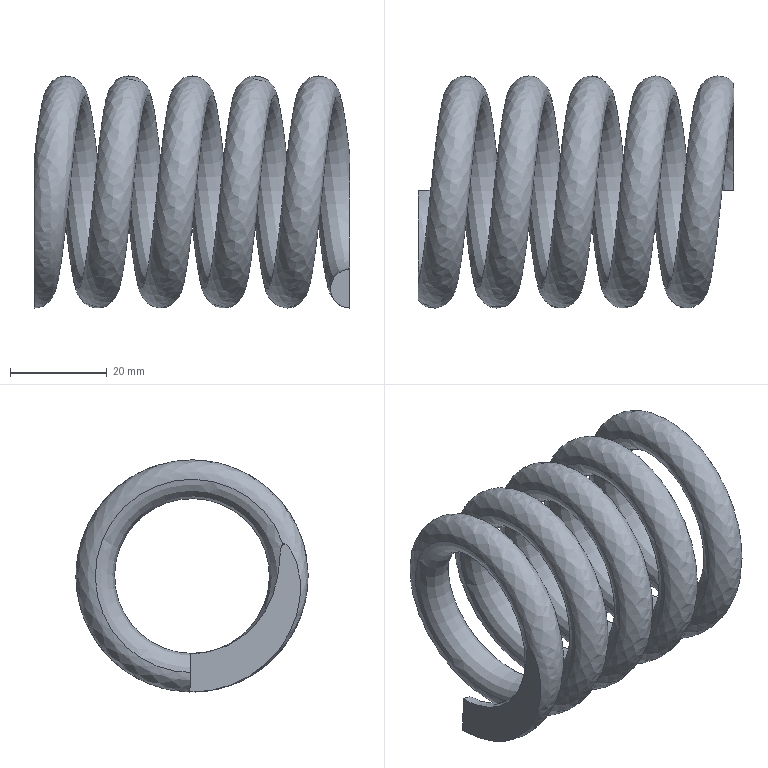Component | SolidWorks | 216InnerTubeAssembly-1_CompressionSpring-1 | 1 solid | 6 faces | volume 30759 mm3 | plane 4 | spline 2